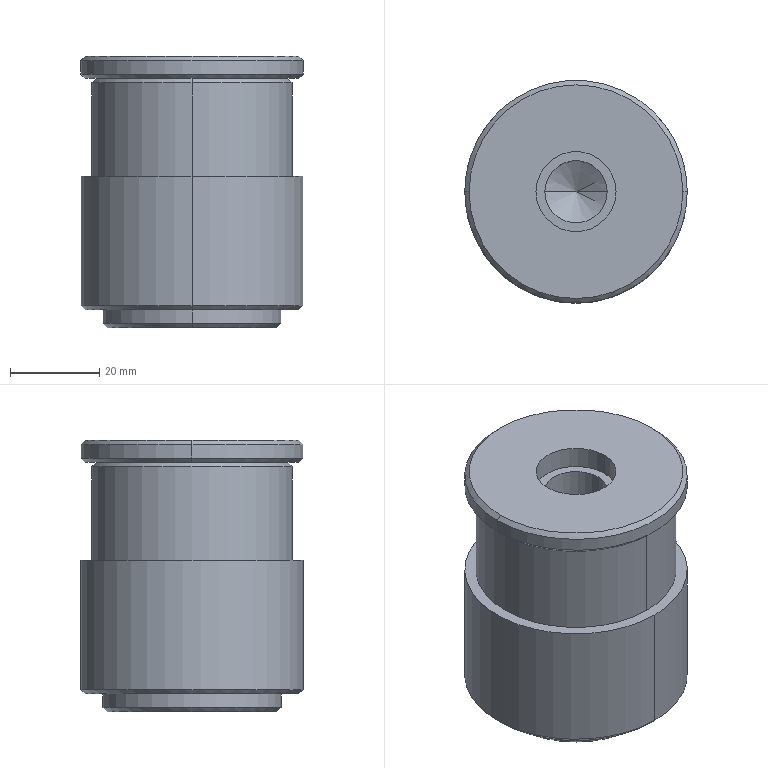Component | SolidWorks | FixedAxis1-1 | 2 solids | 30 faces | box 50 x 50 x 61 mm | volume 102576 mm3 | cone 12 | cylinder 12 | plane 6 | commonest cylinder face diameters 50 x4 14 x2 45 x2 40 x2 18 x2
build123d program:
from build123d import *

# Parameters (mm, degrees)
M16_TAPPED_HOLE1_D     = 14
M16_TAPPED_HOLE1_DEPTH = 28
M16_TAPPED_HOLE1_TIP   = 4.206
CHAMFER1_SIZE          = 1
SKETCH4_R              = 25
SKETCH4_R_2            = 9
BOSS_EXTRUDE1_DEPTH    = 5
CHAMFER2_SIZE          = 1


with BuildPart() as part:
    # Sketch1 → Revolve1 (revolve)
    with BuildSketch(Plane(origin=(0, 0, 0), x_dir=(0, 0, -1), z_dir=(1, 0, 0)), mode=Mode.PRIVATE) as revolve1_sk:
        Polygon((-28, 0), (28, 0), (28, 20), (24, 20), (24, 25), (-6, 25), (-6, 22.5), (-28, 22.5), align=None)
    revolve(revolve1_sk.sketch.rotate(Axis((0, 0, 28), (0, 0, -1)), 180), axis=Axis((0, 0, 28), (0, 0, -1)))

    # M16 Tapped Hole1
    with Locations(Plane.XY.offset(28)):
        with Locations((0, 0)):
            Hole(M16_TAPPED_HOLE1_D / 2, depth=M16_TAPPED_HOLE1_DEPTH)
            with Locations((0, 0, -(M16_TAPPED_HOLE1_DEPTH + M16_TAPPED_HOLE1_TIP / 2))):  # 118° drill point
                Cone(0, M16_TAPPED_HOLE1_D / 2, M16_TAPPED_HOLE1_TIP, mode=Mode.SUBTRACT)

    # Chamfer1
    chamfer1_edges = [part.edges().sort_by_distance(p)[0] for p in [
        (0, 22.5, 28),
        (0, 25, -24),
        (0, 20, -28),
    ]]
    chamfer(chamfer1_edges, length=CHAMFER1_SIZE)


with BuildPart() as body_2:
    # Sketch4 → Boss-Extrude1 (new body)
    with BuildSketch(Plane.XY.offset(28)):
        Circle(SKETCH4_R)
        Circle(SKETCH4_R_2, mode=Mode.SUBTRACT)
    extrude(amount=BOSS_EXTRUDE1_DEPTH)

    # Chamfer2
    chamfer2_edges = [body_2.edges().sort_by_distance(p)[0] for p in [
        (-25, 0, 28),
        (-25, 0, 33),
    ]]
    chamfer(chamfer2_edges, length=CHAMFER2_SIZE)


solid = Compound([part.part, body_2.part])
STEP:
#1=COLOUR_RGB('',0.7922,0.8196,0.9333);
#2=FILL_AREA_STYLE_COLOUR('',#1);
#3=FILL_AREA_STYLE('',(#2));
#4=SURFACE_STYLE_FILL_AREA(#3);
#5=SURFACE_SIDE_STYLE('',(#4));
#6=SURFACE_STYLE_USAGE(.BOTH.,#5);
#7=PRESENTATION_STYLE_ASSIGNMENT((#6));
#8=CARTESIAN_POINT('',(0.,-0.8465,1.102));
#9=VERTEX_POINT('',#8);
#10=CARTESIAN_POINT('',(0.,0.8465,1.102));
#11=VERTEX_POINT('',#10);
#12=CARTESIAN_POINT('',(0.,-0.,1.102));
#13=DIRECTION('',(0.,-0.,1.));
#14=DIRECTION('',(0.,1.,0.));
#15=AXIS2_PLACEMENT_3D('',#12,#13,#14);
#16=CIRCLE('',#15,0.8465);
#17=EDGE_CURVE('',#9,#11,#16,.T.);
#18=ORIENTED_EDGE('',*,*,#17,.F.);
#19=CARTESIAN_POINT('',(0.,-0.8858,1.063));
#20=VERTEX_POINT('',#19);
#21=CARTESIAN_POINT('',(0.,-0.8465,1.102));
#22=DIRECTION('',(0.,-0.7071,-0.7071));
#23=VECTOR('',#22,39.37);
#24=LINE('',#21,#23);
#25=EDGE_CURVE('',#9,#20,#24,.T.);
#26=ORIENTED_EDGE('',*,*,#25,.T.);
#27=CARTESIAN_POINT('',(0.,0.8858,1.063));
#28=VERTEX_POINT('',#27);
#29=CARTESIAN_POINT('',(0.,-0.,1.063));
#30=DIRECTION('',(0.,0.,-1.));
#31=DIRECTION('',(0.,1.,0.));
#32=AXIS2_PLACEMENT_3D('',#29,#30,#31);
#33=CIRCLE('',#32,0.8858);
#34=EDGE_CURVE('',#28,#20,#33,.T.);
#35=ORIENTED_EDGE('',*,*,#34,.F.);
#36=CARTESIAN_POINT('',(0.,0.8465,1.102));
#37=DIRECTION('',(0.,0.7071,-0.7071));
#38=VECTOR('',#37,39.37);
#39=LINE('',#36,#38);
#40=EDGE_CURVE('',#11,#28,#39,.T.);
#41=ORIENTED_EDGE('',*,*,#40,.F.);
#42=EDGE_LOOP('',(#18,#26,#35,#41));
#43=FACE_OUTER_BOUND('',#42,.T.);
#44=CARTESIAN_POINT('',(0.,-0.,1.102));
#45=DIRECTION('',(0.,0.,-1.));
#46=DIRECTION('',(0.,1.,0.));
#47=AXIS2_PLACEMENT_3D('',#44,#45,#46);
#48=CONICAL_SURFACE('',#47,0.8465,0.7854);
#49=ADVANCED_FACE('',(#43),#48,.T.);
#50=CARTESIAN_POINT('',(0.,0.748,-1.102));
#51=VERTEX_POINT('',#50);
#52=CARTESIAN_POINT('',(0.,-0.748,-1.102));
#53=VERTEX_POINT('',#52);
#54=CARTESIAN_POINT('',(0.,-0.,-1.102));
#55=DIRECTION('',(0.,0.,-1.));
#56=DIRECTION('',(0.,-1.,-0.));
#57=AXIS2_PLACEMENT_3D('',#54,#55,#56);
#58=CIRCLE('',#57,0.748);
#59=EDGE_CURVE('',#51,#53,#58,.T.);
#60=ORIENTED_EDGE('',*,*,#59,.F.);
#61=CARTESIAN_POINT('',(0.,0.7874,-1.063));
#62=VERTEX_POINT('',#61);
#63=CARTESIAN_POINT('',(0.,0.7874,-1.063));
#64=DIRECTION('',(0.,0.7071,0.7071));
#65=VECTOR('',#64,39.37);
#66=LINE('',#63,#65);
#67=EDGE_CURVE('',#51,#62,#66,.T.);
#68=ORIENTED_EDGE('',*,*,#67,.T.);
#69=CARTESIAN_POINT('',(0.,-0.7874,-1.063));
#70=VERTEX_POINT('',#69);
#71=CARTESIAN_POINT('',(0.,-0.,-1.063));
#72=DIRECTION('',(0.,-0.,1.));
#73=DIRECTION('',(0.,-1.,-0.));
#74=AXIS2_PLACEMENT_3D('',#71,#72,#73);
#75=CIRCLE('',#74,0.7874);
#76=EDGE_CURVE('',#70,#62,#75,.T.);
#77=ORIENTED_EDGE('',*,*,#76,.F.);
#78=CARTESIAN_POINT('',(0.,-0.7874,-1.063));
#79=DIRECTION('',(0.,-0.7071,0.7071));
#80=VECTOR('',#79,39.37);
#81=LINE('',#78,#80);
#82=EDGE_CURVE('',#53,#70,#81,.T.);
#83=ORIENTED_EDGE('',*,*,#82,.F.);
#84=EDGE_LOOP('',(#60,#68,#77,#83));
#85=FACE_OUTER_BOUND('',#84,.T.);
#86=CARTESIAN_POINT('',(0.,-0.,-1.063));
#87=DIRECTION('',(0.,-0.,1.));
#88=DIRECTION('',(0.,-1.,-0.));
#89=AXIS2_PLACEMENT_3D('',#86,#87,#88);
#90=CONICAL_SURFACE('',#89,0.7874,0.7854);
#91=ADVANCED_FACE('',(#85),#90,.T.);
#92=CARTESIAN_POINT('',(0.,0.9449,-0.9449));
#93=VERTEX_POINT('',#92);
#94=CARTESIAN_POINT('',(0.,-0.9449,-0.9449));
#95=VERTEX_POINT('',#94);
#96=CARTESIAN_POINT('',(0.,-0.,-0.9449));
#97=DIRECTION('',(0.,0.,-1.));
#98=DIRECTION('',(0.,-1.,-0.));
#99=AXIS2_PLACEMENT_3D('',#96,#97,#98);
#100=CIRCLE('',#99,0.9449);
#101=EDGE_CURVE('',#93,#95,#100,.T.);
#102=ORIENTED_EDGE('',*,*,#101,.F.);
#103=CARTESIAN_POINT('',(0.,0.9843,-0.9055));
#104=VERTEX_POINT('',#103);
#105=CARTESIAN_POINT('',(0.,0.9843,-0.9055));
#106=DIRECTION('',(0.,0.7071,0.7071));
#107=VECTOR('',#106,39.37);
#108=LINE('',#105,#107);
#109=EDGE_CURVE('',#93,#104,#108,.T.);
#110=ORIENTED_EDGE('',*,*,#109,.T.);
#111=CARTESIAN_POINT('',(0.,-0.9843,-0.9055));
#112=VERTEX_POINT('',#111);
#113=CARTESIAN_POINT('',(0.,-0.,-0.9055));
#114=DIRECTION('',(0.,-0.,1.));
#115=DIRECTION('',(0.,-1.,-0.));
#116=AXIS2_PLACEMENT_3D('',#113,#114,#115);
#117=CIRCLE('',#116,0.9843);
#118=EDGE_CURVE('',#112,#104,#117,.T.);
#119=ORIENTED_EDGE('',*,*,#118,.F.);
#120=CARTESIAN_POINT('',(0.,-0.9843,-0.9055));
#121=DIRECTION('',(0.,-0.7071,0.7071));
#122=VECTOR('',#121,39.37);
#123=LINE('',#120,#122);
#124=EDGE_CURVE('',#95,#112,#123,.T.);
#125=ORIENTED_EDGE('',*,*,#124,.F.);
#126=EDGE_LOOP('',(#102,#110,#119,#125));
#127=FACE_OUTER_BOUND('',#126,.T.);
#128=CARTESIAN_POINT('',(0.,-0.,-0.9055));
#129=DIRECTION('',(0.,-0.,1.));
#130=DIRECTION('',(0.,-1.,-0.));
#131=AXIS2_PLACEMENT_3D('',#128,#129,#130);
#132=CONICAL_SURFACE('',#131,0.9843,0.7854);
#133=ADVANCED_FACE('',(#127),#132,.T.);
#134=CARTESIAN_POINT('',(-0.2756,0.,-0.));
#135=VERTEX_POINT('',#134);
#136=CARTESIAN_POINT('',(0.2756,0.,-0.));
#137=VERTEX_POINT('',#136);
#138=CARTESIAN_POINT('',(0.,0.,-0.));
#139=DIRECTION('',(0.,0.,1.));
#140=DIRECTION('',(1.,0.,0.));
#141=AXIS2_PLACEMENT_3D('',#138,#139,#140);
#142=CIRCLE('',#141,0.2756);
#143=EDGE_CURVE('',#135,#137,#142,.T.);
#144=ORIENTED_EDGE('',*,*,#143,.F.);
#145=CARTESIAN_POINT('',(-0.2756,0.,1.102));
#146=VERTEX_POINT('',#145);
#147=CARTESIAN_POINT('',(-0.2756,0.,1.102));
#148=DIRECTION('',(0.,0.,1.));
#149=VECTOR('',#148,39.37);
#150=LINE('',#147,#149);
#151=EDGE_CURVE('',#135,#146,#150,.T.);
#152=ORIENTED_EDGE('',*,*,#151,.T.);
#153=CARTESIAN_POINT('',(0.2756,0.,1.102));
#154=VERTEX_POINT('',#153);
#155=CARTESIAN_POINT('',(0.,0.,1.102));
#156=DIRECTION('',(0.,0.,1.));
#157=DIRECTION('',(1.,0.,0.));
#158=AXIS2_PLACEMENT_3D('',#155,#156,#157);
#159=CIRCLE('',#158,0.2756);
#160=EDGE_CURVE('',#146,#154,#159,.T.);
#161=ORIENTED_EDGE('',*,*,#160,.T.);
#162=CARTESIAN_POINT('',(0.2756,0.,1.102));
#163=DIRECTION('',(0.,0.,1.));
#164=VECTOR('',#163,39.37);
#165=LINE('',#162,#164);
#166=EDGE_CURVE('',#137,#154,#165,.T.);
#167=ORIENTED_EDGE('',*,*,#166,.F.);
#168=EDGE_LOOP('',(#144,#152,#161,#167));
#169=FACE_OUTER_BOUND('',#168,.T.);
#170=CARTESIAN_POINT('',(0.,0.,1.102));
#171=DIRECTION('',(0.,0.,1.));
#172=DIRECTION('',(1.,0.,0.));
#173=AXIS2_PLACEMENT_3D('',#170,#171,#172);
#174=CYLINDRICAL_SURFACE('',#173,0.2756);
#175=ADVANCED_FACE('',(#169),#174,.F.);
#176=CARTESIAN_POINT('',(-0.,0.,-0.1656));
#177=VERTEX_POINT('',#176);
#178=CARTESIAN_POINT('',(0.2756,0.,-0.));
#179=DIRECTION('',(0.8572,0.,0.515));
#180=VECTOR('',#179,39.37);
#181=LINE('',#178,#180);
#182=EDGE_CURVE('',#177,#137,#181,.T.);
#183=ORIENTED_EDGE('',*,*,#182,.F.);
#184=CARTESIAN_POINT('',(-0.2756,0.,-0.));
#185=DIRECTION('',(-0.8572,0.,0.515));
#186=VECTOR('',#185,39.37);
#187=LINE('',#184,#186);
#188=EDGE_CURVE('',#177,#135,#187,.T.);
#189=ORIENTED_EDGE('',*,*,#188,.T.);
#190=ORIENTED_EDGE('',*,*,#143,.T.);
#191=EDGE_LOOP('',(#183,#189,#190));
#192=FACE_OUTER_BOUND('',#191,.T.);
#193=CARTESIAN_POINT('',(0.,0.,-0.));
#194=DIRECTION('',(0.,0.,1.));
#195=DIRECTION('',(1.,0.,0.));
#196=AXIS2_PLACEMENT_3D('',#193,#194,#195);
#197=CONICAL_SURFACE('',#196,0.2756,1.03);
#198=ADVANCED_FACE('',(#192),#197,.F.);
#199=CARTESIAN_POINT('',(0.,-0.8858,0.2362));
#200=VERTEX_POINT('',#199);
#201=CARTESIAN_POINT('',(0.,0.8858,0.2362));
#202=VERTEX_POINT('',#201);
#203=CARTESIAN_POINT('',(0.,-0.,0.2362));
#204=DIRECTION('',(0.,-0.,1.));
#205=DIRECTION('',(0.,-1.,-0.));
#206=AXIS2_PLACEMENT_3D('',#203,#204,#205);
#207=CIRCLE('',#206,0.8858);
#208=EDGE_CURVE('',#200,#202,#207,.T.);
#209=ORIENTED_EDGE('',*,*,#208,.T.);
#210=CARTESIAN_POINT('',(0.,0.8858,1.102));
#211=DIRECTION('',(0.,-0.,1.));
#212=VECTOR('',#211,39.37);
#213=LINE('',#210,#212);
#214=EDGE_CURVE('',#202,#28,#213,.T.);
#215=ORIENTED_EDGE('',*,*,#214,.T.);
#216=ORIENTED_EDGE('',*,*,#34,.T.);
#217=CARTESIAN_POINT('',(0.,-0.8858,1.102));
#218=DIRECTION('',(0.,-0.,1.));
#219=VECTOR('',#218,39.37);
#220=LINE('',#217,#219);
#221=EDGE_CURVE('',#200,#20,#220,.T.);
#222=ORIENTED_EDGE('',*,*,#221,.F.);
#223=EDGE_LOOP('',(#209,#215,#216,#222));
#224=FACE_OUTER_BOUND('',#223,.T.);
#225=CARTESIAN_POINT('',(0.,-0.,1.102));
#226=DIRECTION('',(0.,-0.,1.));
#227=DIRECTION('',(0.,-1.,-0.));
#228=AXIS2_PLACEMENT_3D('',#225,#226,#227);
#229=CYLINDRICAL_SURFACE('',#228,0.8858);
#230=ADVANCED_FACE('',(#224),#229,.T.);
#231=ORIENTED_EDGE('',*,*,#118,.T.);
#232=CARTESIAN_POINT('',(0.,0.9843,0.2362));
#233=VERTEX_POINT('',#232);
#234=CARTESIAN_POINT('',(0.,0.9843,1.102));
#235=DIRECTION('',(0.,-0.,1.));
#236=VECTOR('',#235,39.37);
#237=LINE('',#234,#236);
#238=EDGE_CURVE('',#104,#233,#237,.T.);
#239=ORIENTED_EDGE('',*,*,#238,.T.);
#240=CARTESIAN_POINT('',(0.,-0.9843,0.2362));
#241=VERTEX_POINT('',#240);
#242=CARTESIAN_POINT('',(0.,-0.,0.2362));
#243=DIRECTION('',(0.,-0.,1.));
#244=DIRECTION('',(0.,-1.,-0.));
#245=AXIS2_PLACEMENT_3D('',#242,#243,#244);
#246=CIRCLE('',#245,0.9843);
#247=EDGE_CURVE('',#241,#233,#246,.T.);
#248=ORIENTED_EDGE('',*,*,#247,.F.);
#249=CARTESIAN_POINT('',(0.,-0.9843,1.102));
#250=DIRECTION('',(0.,-0.,1.));
#251=VECTOR('',#250,39.37);
#252=LINE('',#249,#251);
#253=EDGE_CURVE('',#112,#241,#252,.T.);
#254=ORIENTED_EDGE('',*,*,#253,.F.);
#255=EDGE_LOOP('',(#231,#239,#248,#254));
#256=FACE_OUTER_BOUND('',#255,.T.);
#257=CARTESIAN_POINT('',(0.,-0.,1.102));
#258=DIRECTION('',(0.,-0.,1.));
#259=DIRECTION('',(0.,-1.,-0.));
#260=AXIS2_PLACEMENT_3D('',#257,#258,#259);
#261=CYLINDRICAL_SURFACE('',#260,0.9843);
#262=ADVANCED_FACE('',(#256),#261,.T.);
#263=ORIENTED_EDGE('',*,*,#76,.T.);
#264=CARTESIAN_POINT('',(0.,0.7874,-0.9449));
#265=VERTEX_POINT('',#264);
#266=CARTESIAN_POINT('',(0.,0.7874,1.102));
#267=DIRECTION('',(0.,-0.,1.));
#268=VECTOR('',#267,39.37);
#269=LINE('',#266,#268);
#270=EDGE_CURVE('',#62,#265,#269,.T.);
#271=ORIENTED_EDGE('',*,*,#270,.T.);
#272=CARTESIAN_POINT('',(0.,-0.7874,-0.9449));
#273=VERTEX_POINT('',#272);
#274=CARTESIAN_POINT('',(0.,-0.,-0.9449));
#275=DIRECTION('',(0.,-0.,1.));
#276=DIRECTION('',(0.,-1.,-0.));
#277=AXIS2_PLACEMENT_3D('',#274,#275,#276);
#278=CIRCLE('',#277,0.7874);
#279=EDGE_CURVE('',#273,#265,#278,.T.);
#280=ORIENTED_EDGE('',*,*,#279,.F.);
#281=CARTESIAN_POINT('',(0.,-0.7874,1.102));
#282=DIRECTION('',(0.,-0.,1.));
#283=VECTOR('',#282,39.37);
#284=LINE('',#281,#283);
#285=EDGE_CURVE('',#70,#273,#284,.T.);
#286=ORIENTED_EDGE('',*,*,#285,.F.);
#287=EDGE_LOOP('',(#263,#271,#280,#286));
#288=FACE_OUTER_BOUND('',#287,.T.);
#289=CARTESIAN_POINT('',(0.,-0.,1.102));
#290=DIRECTION('',(0.,-0.,1.));
#291=DIRECTION('',(0.,-1.,-0.));
#292=AXIS2_PLACEMENT_3D('',#289,#290,#291);
#293=CYLINDRICAL_SURFACE('',#292,0.7874);
#294=ADVANCED_FACE('',(#288),#293,.T.);
#295=CARTESIAN_POINT('',(0.,-0.,1.102));
#296=DIRECTION('',(0.,-0.,1.));
#297=DIRECTION('',(0.,1.,0.));
#298=AXIS2_PLACEMENT_3D('',#295,#296,#297);
#299=CIRCLE('',#298,0.8465);
#300=EDGE_CURVE('',#11,#9,#299,.T.);
#301=ORIENTED_EDGE('',*,*,#300,.T.);
#302=ORIENTED_EDGE('',*,*,#17,.T.);
#303=EDGE_LOOP('',(#301,#302));
#304=FACE_OUTER_BOUND('',#303,.T.);
#305=CARTESIAN_POINT('',(0.,0.,1.102));
#306=DIRECTION('',(0.,0.,1.));
#307=DIRECTION('',(1.,0.,0.));
#308=AXIS2_PLACEMENT_3D('',#305,#306,#307);
#309=CIRCLE('',#308,0.2756);
#310=EDGE_CURVE('',#154,#146,#309,.T.);
#311=ORIENTED_EDGE('',*,*,#310,.F.);
#312=ORIENTED_EDGE('',*,*,#160,.F.);
#313=EDGE_LOOP('',(#311,#312));
#314=FACE_BOUND('',#313,.T.);
#315=CARTESIAN_POINT('',(0.,0.8858,1.102));
#316=DIRECTION('',(0.,0.,-1.));
#317=DIRECTION('',(0.,1.,0.));
#318=AXIS2_PLACEMENT_3D('',#315,#316,#317);
#319=PLANE('',#318);
#320=ADVANCED_FACE('',(#304,#314),#319,.F.);
#321=CARTESIAN_POINT('',(0.,-0.,-1.102));
#322=DIRECTION('',(0.,0.,-1.));
#323=DIRECTION('',(0.,-1.,-0.));
#324=AXIS2_PLACEMENT_3D('',#321,#322,#323);
#325=CIRCLE('',#324,0.748);
#326=EDGE_CURVE('',#53,#51,#325,.T.);
#327=ORIENTED_EDGE('',*,*,#326,.T.);
#328=ORIENTED_EDGE('',*,*,#59,.T.);
#329=EDGE_LOOP('',(#327,#328));
#330=FACE_OUTER_BOUND('',#329,.T.);
#331=CARTESIAN_POINT('',(0.,-0.,-1.102));
#332=DIRECTION('',(0.,-0.,1.));
#333=DIRECTION('',(0.,-1.,-0.));
#334=AXIS2_PLACEMENT_3D('',#331,#332,#333);
#335=PLANE('',#334);
#336=ADVANCED_FACE('',(#330),#335,.F.);
#337=ORIENTED_EDGE('',*,*,#270,.F.);
#338=CARTESIAN_POINT('',(0.,-0.,-1.063));
#339=DIRECTION('',(0.,-0.,1.));
#340=DIRECTION('',(0.,-1.,-0.));
#341=AXIS2_PLACEMENT_3D('',#338,#339,#340);
#342=CIRCLE('',#341,0.7874);
#343=EDGE_CURVE('',#62,#70,#342,.T.);
#344=ORIENTED_EDGE('',*,*,#343,.T.);
#345=ORIENTED_EDGE('',*,*,#285,.T.);
#346=CARTESIAN_POINT('',(0.,-0.,-0.9449));
#347=DIRECTION('',(0.,-0.,1.));
#348=DIRECTION('',(0.,-1.,-0.));
#349=AXIS2_PLACEMENT_3D('',#346,#347,#348);
#350=CIRCLE('',#349,0.7874);
#351=EDGE_CURVE('',#265,#273,#350,.T.);
#352=ORIENTED_EDGE('',*,*,#351,.F.);
#353=EDGE_LOOP('',(#337,#344,#345,#352));
#354=FACE_OUTER_BOUND('',#353,.T.);
#355=CARTESIAN_POINT('',(0.,-0.,1.102));
#356=DIRECTION('',(0.,-0.,1.));
#357=DIRECTION('',(0.,-1.,-0.));
#358=AXIS2_PLACEMENT_3D('',#355,#356,#357);
#359=CYLINDRICAL_SURFACE('',#358,0.7874);
#360=ADVANCED_FACE('',(#354),#359,.T.);
#361=CARTESIAN_POINT('',(0.,-0.,-0.9449));
#362=DIRECTION('',(0.,0.,-1.));
#363=DIRECTION('',(0.,-1.,-0.));
#364=AXIS2_PLACEMENT_3D('',#361,#362,#363);
#365=CIRCLE('',#364,0.9449);
#366=EDGE_CURVE('',#95,#93,#365,.T.);
#367=ORIENTED_EDGE('',*,*,#366,.T.);
#368=ORIENTED_EDGE('',*,*,#101,.T.);
#369=EDGE_LOOP('',(#367,#368));
#370=FACE_OUTER_BOUND('',#369,.T.);
#371=ORIENTED_EDGE('',*,*,#279,.T.);
#372=ORIENTED_EDGE('',*,*,#351,.T.);
#373=EDGE_LOOP('',(#371,#372));
#374=FACE_BOUND('',#373,.T.);
#375=CARTESIAN_POINT('',(0.,0.7874,-0.9449));
#376=DIRECTION('',(0.,-0.,1.));
#377=DIRECTION('',(0.,-1.,-0.));
#378=AXIS2_PLACEMENT_3D('',#375,#376,#377);
#379=PLANE('',#378);
#380=ADVANCED_FACE('',(#370,#374),#379,.F.);
#381=ORIENTED_EDGE('',*,*,#238,.F.);
#382=CARTESIAN_POINT('',(0.,-0.,-0.9055));
#383=DIRECTION('',(0.,-0.,1.));
#384=DIRECTION('',(0.,-1.,-0.));
#385=AXIS2_PLACEMENT_3D('',#382,#383,#384);
#386=CIRCLE('',#385,0.9843);
#387=EDGE_CURVE('',#104,#112,#386,.T.);
#388=ORIENTED_EDGE('',*,*,#387,.T.);
#389=ORIENTED_EDGE('',*,*,#253,.T.);
#390=CARTESIAN_POINT('',(0.,-0.,0.2362));
#391=DIRECTION('',(0.,-0.,1.));
#392=DIRECTION('',(0.,-1.,-0.));
#393=AXIS2_PLACEMENT_3D('',#390,#391,#392);
#394=CIRCLE('',#393,0.9843);
#395=EDGE_CURVE('',#233,#241,#394,.T.);
#396=ORIENTED_EDGE('',*,*,#395,.F.);
#397=EDGE_LOOP('',(#381,#388,#389,#396));
#398=FACE_OUTER_BOUND('',#397,.T.);
#399=CARTESIAN_POINT('',(0.,-0.,1.102));
#400=DIRECTION('',(0.,-0.,1.));
#401=DIRECTION('',(0.,-1.,-0.));
#402=AXIS2_PLACEMENT_3D('',#399,#400,#401);
#403=CYLINDRICAL_SURFACE('',#402,0.9843);
#404=ADVANCED_FACE('',(#398),#403,.T.);
#405=ORIENTED_EDGE('',*,*,#208,.F.);
#406=CARTESIAN_POINT('',(0.,-0.,0.2362));
#407=DIRECTION('',(0.,-0.,1.));
#408=DIRECTION('',(0.,-1.,-0.));
#409=AXIS2_PLACEMENT_3D('',#406,#407,#408);
#410=CIRCLE('',#409,0.8858);
#411=EDGE_CURVE('',#202,#200,#410,.T.);
#412=ORIENTED_EDGE('',*,*,#411,.F.);
#413=EDGE_LOOP('',(#405,#412));
#414=FACE_BOUND('',#413,.T.);
#415=ORIENTED_EDGE('',*,*,#247,.T.);
#416=ORIENTED_EDGE('',*,*,#395,.T.);
#417=EDGE_LOOP('',(#415,#416));
#418=FACE_OUTER_BOUND('',#417,.T.);
#419=CARTESIAN_POINT('',(0.,0.9843,0.2362));
#420=DIRECTION('',(0.,0.,-1.));
#421=DIRECTION('',(0.,1.,0.));
#422=AXIS2_PLACEMENT_3D('',#419,#420,#421);
#423=PLANE('',#422);
#424=ADVANCED_FACE('',(#414,#418),#423,.F.);
#425=ORIENTED_EDGE('',*,*,#214,.F.);
#426=ORIENTED_EDGE('',*,*,#411,.T.);
#427=ORIENTED_EDGE('',*,*,#221,.T.);
#428=CARTESIAN_POINT('',(0.,-0.,1.063));
#429=DIRECTION('',(0.,0.,-1.));
#430=DIRECTION('',(0.,1.,0.));
#431=AXIS2_PLACEMENT_3D('',#428,#429,#430);
#432=CIRCLE('',#431,0.8858);
#433=EDGE_CURVE('',#20,#28,#432,.T.);
#434=ORIENTED_EDGE('',*,*,#433,.T.);
#435=EDGE_LOOP('',(#425,#426,#427,#434));
#436=FACE_OUTER_BOUND('',#435,.T.);
#437=CARTESIAN_POINT('',(0.,-0.,1.102));
#438=DIRECTION('',(0.,-0.,1.));
#439=DIRECTION('',(0.,-1.,-0.));
#440=AXIS2_PLACEMENT_3D('',#437,#438,#439);
#441=CYLINDRICAL_SURFACE('',#440,0.8858);
#442=ADVANCED_FACE('',(#436),#441,.T.);
#443=ORIENTED_EDGE('',*,*,#188,.F.);
#444=ORIENTED_EDGE('',*,*,#182,.T.);
#445=CARTESIAN_POINT('',(0.,0.,-0.));
#446=DIRECTION('',(0.,0.,1.));
#447=DIRECTION('',(1.,0.,0.));
#448=AXIS2_PLACEMENT_3D('',#445,#446,#447);
#449=CIRCLE('',#448,0.2756);
#450=EDGE_CURVE('',#137,#135,#449,.T.);
#451=ORIENTED_EDGE('',*,*,#450,.T.);
#452=EDGE_LOOP('',(#443,#444,#451));
#453=FACE_OUTER_BOUND('',#452,.T.);
#454=CARTESIAN_POINT('',(0.,0.,-0.));
#455=DIRECTION('',(0.,0.,1.));
#456=DIRECTION('',(1.,0.,0.));
#457=AXIS2_PLACEMENT_3D('',#454,#455,#456);
#458=CONICAL_SURFACE('',#457,0.2756,1.03);
#459=ADVANCED_FACE('',(#453),#458,.F.);
#460=ORIENTED_EDGE('',*,*,#151,.F.);
#461=ORIENTED_EDGE('',*,*,#450,.F.);
#462=ORIENTED_EDGE('',*,*,#166,.T.);
#463=ORIENTED_EDGE('',*,*,#310,.T.);
#464=EDGE_LOOP('',(#460,#461,#462,#463));
#465=FACE_OUTER_BOUND('',#464,.T.);
#466=CARTESIAN_POINT('',(0.,0.,1.102));
#467=DIRECTION('',(0.,0.,1.));
#468=DIRECTION('',(1.,0.,0.));
#469=AXIS2_PLACEMENT_3D('',#466,#467,#468);
#470=CYLINDRICAL_SURFACE('',#469,0.2756);
#471=ADVANCED_FACE('',(#465),#470,.F.);
#472=ORIENTED_EDGE('',*,*,#109,.F.);
#473=ORIENTED_EDGE('',*,*,#366,.F.);
#474=ORIENTED_EDGE('',*,*,#124,.T.);
#475=ORIENTED_EDGE('',*,*,#387,.F.);
#476=EDGE_LOOP('',(#472,#473,#474,#475));
#477=FACE_OUTER_BOUND('',#476,.T.);
#478=CARTESIAN_POINT('',(0.,-0.,-0.9055));
#479=DIRECTION('',(0.,-0.,1.));
#480=DIRECTION('',(0.,-1.,-0.));
#481=AXIS2_PLACEMENT_3D('',#478,#479,#480);
#482=CONICAL_SURFACE('',#481,0.9843,0.7854);
#483=ADVANCED_FACE('',(#477),#482,.T.);
#484=ORIENTED_EDGE('',*,*,#67,.F.);
#485=ORIENTED_EDGE('',*,*,#326,.F.);
#486=ORIENTED_EDGE('',*,*,#82,.T.);
#487=ORIENTED_EDGE('',*,*,#343,.F.);
#488=EDGE_LOOP('',(#484,#485,#486,#487));
#489=FACE_OUTER_BOUND('',#488,.T.);
#490=CARTESIAN_POINT('',(0.,-0.,-1.063));
#491=DIRECTION('',(0.,-0.,1.));
#492=DIRECTION('',(0.,-1.,-0.));
#493=AXIS2_PLACEMENT_3D('',#490,#491,#492);
#494=CONICAL_SURFACE('',#493,0.7874,0.7854);
#495=ADVANCED_FACE('',(#489),#494,.T.);
#496=ORIENTED_EDGE('',*,*,#25,.F.);
#497=ORIENTED_EDGE('',*,*,#300,.F.);
#498=ORIENTED_EDGE('',*,*,#40,.T.);
#499=ORIENTED_EDGE('',*,*,#433,.F.);
#500=EDGE_LOOP('',(#496,#497,#498,#499));
#501=FACE_OUTER_BOUND('',#500,.T.);
#502=CARTESIAN_POINT('',(0.,-0.,1.102));
#503=DIRECTION('',(0.,0.,-1.));
#504=DIRECTION('',(0.,1.,0.));
#505=AXIS2_PLACEMENT_3D('',#502,#503,#504);
#506=CONICAL_SURFACE('',#505,0.8465,0.7854);
#507=ADVANCED_FACE('',(#501),#506,.T.);
#508=CLOSED_SHELL('',(#49,#91,#133,#175,#198,#230,#262,#294,#320,#336,#360,#380,#404,#424,#442,#459,#471,#483,#495,#507));
#509=MANIFOLD_SOLID_BREP('',#508);
#510=STYLED_ITEM('',(#7),#509);
#511=PRESENTATION_LAYER_ASSIGNMENT('','',(#510));
#512=(LENGTH_UNIT()NAMED_UNIT(*)SI_UNIT($,.METRE.));
#513=LENGTH_MEASURE_WITH_UNIT(LENGTH_MEASURE(0.0254),#512);
#514=DIMENSIONAL_EXPONENTS(1.,0.,0.,0.,0.,0.,0.);
#515=(CONVERSION_BASED_UNIT('',#513)LENGTH_UNIT()NAMED_UNIT(#514));
#516=UNCERTAINTY_MEASURE_WITH_UNIT(LENGTH_MEASURE(0.00001),#515,'','');
#517=(NAMED_UNIT(*)PLANE_ANGLE_UNIT()SI_UNIT($,.RADIAN.));
#518=(NAMED_UNIT(*)SI_UNIT($,.STERADIAN.)SOLID_ANGLE_UNIT());
#519=(GEOMETRIC_REPRESENTATION_CONTEXT(3)GLOBAL_UNCERTAINTY_ASSIGNED_CONTEXT((#516))GLOBAL_UNIT_ASSIGNED_CONTEXT((#515,#517,#518))REPRESENTATION_CONTEXT('',''));
#520=MECHANICAL_DESIGN_GEOMETRIC_PRESENTATION_REPRESENTATION('',(#510),#519);
#521=COLOUR_RGB('',0.7922,0.8196,0.9333);
#522=FILL_AREA_STYLE_COLOUR('',#521);
#523=FILL_AREA_STYLE('',(#522));
#524=SURFACE_STYLE_FILL_AREA(#523);
#525=SURFACE_SIDE_STYLE('',(#524));
#526=SURFACE_STYLE_USAGE(.BOTH.,#525);
#527=PRESENTATION_STYLE_ASSIGNMENT((#526));
#528=CARTESIAN_POINT('',(0.9449,0.,1.299));
#529=VERTEX_POINT('',#528);
#530=CARTESIAN_POINT('',(-0.9449,0.,1.299));
#531=VERTEX_POINT('',#530);
#532=CARTESIAN_POINT('',(0.,0.,1.299));
#533=DIRECTION('',(0.,0.,1.));
#534=DIRECTION('',(1.,0.,0.));
#535=AXIS2_PLACEMENT_3D('',#532,#533,#534);
#536=CIRCLE('',#535,0.9449);
#537=EDGE_CURVE('',#529,#531,#536,.T.);
#538=ORIENTED_EDGE('',*,*,#537,.F.);
#539=CARTESIAN_POINT('',(0.9843,0.,1.26));
#540=VERTEX_POINT('',#539);
#541=CARTESIAN_POINT('',(0.9449,0.,1.299));
#542=DIRECTION('',(0.7071,0.,-0.7071));
#543=VECTOR('',#542,39.37);
#544=LINE('',#541,#543);
#545=EDGE_CURVE('',#529,#540,#544,.T.);
#546=ORIENTED_EDGE('',*,*,#545,.T.);
#547=CARTESIAN_POINT('',(-0.9843,0.,1.26));
#548=VERTEX_POINT('',#547);
#549=CARTESIAN_POINT('',(0.,0.,1.26));
#550=DIRECTION('',(0.,0.,-1.));
#551=DIRECTION('',(1.,0.,0.));
#552=AXIS2_PLACEMENT_3D('',#549,#550,#551);
#553=CIRCLE('',#552,0.9843);
#554=EDGE_CURVE('',#548,#540,#553,.T.);
#555=ORIENTED_EDGE('',*,*,#554,.F.);
#556=CARTESIAN_POINT('',(-0.9449,0.,1.299));
#557=DIRECTION('',(-0.7071,0.,-0.7071));
#558=VECTOR('',#557,39.37);
#559=LINE('',#556,#558);
#560=EDGE_CURVE('',#531,#548,#559,.T.);
#561=ORIENTED_EDGE('',*,*,#560,.F.);
#562=EDGE_LOOP('',(#538,#546,#555,#561));
#563=FACE_OUTER_BOUND('',#562,.T.);
#564=CARTESIAN_POINT('',(0.,0.,1.299));
#565=DIRECTION('',(0.,0.,-1.));
#566=DIRECTION('',(-1.,0.,0.));
#567=AXIS2_PLACEMENT_3D('',#564,#565,#566);
#568=CONICAL_SURFACE('',#567,0.9449,0.7854);
#569=ADVANCED_FACE('',(#563),#568,.T.);
#570=CARTESIAN_POINT('',(-0.9449,0.,1.102));
#571=VERTEX_POINT('',#570);
#572=CARTESIAN_POINT('',(0.9449,0.,1.102));
#573=VERTEX_POINT('',#572);
#574=CARTESIAN_POINT('',(0.,0.,1.102));
#575=DIRECTION('',(0.,0.,-1.));
#576=DIRECTION('',(1.,0.,0.));
#577=AXIS2_PLACEMENT_3D('',#574,#575,#576);
#578=CIRCLE('',#577,0.9449);
#579=EDGE_CURVE('',#571,#573,#578,.T.);
#580=ORIENTED_EDGE('',*,*,#579,.F.);
#581=CARTESIAN_POINT('',(-0.9843,0.,1.142));
#582=VERTEX_POINT('',#581);
#583=CARTESIAN_POINT('',(-0.9843,0.,1.142));
#584=DIRECTION('',(-0.7071,0.,0.7071));
#585=VECTOR('',#584,39.37);
#586=LINE('',#583,#585);
#587=EDGE_CURVE('',#571,#582,#586,.T.);
#588=ORIENTED_EDGE('',*,*,#587,.T.);
#589=CARTESIAN_POINT('',(0.9843,0.,1.142));
#590=VERTEX_POINT('',#589);
#591=CARTESIAN_POINT('',(0.,0.,1.142));
#592=DIRECTION('',(0.,0.,1.));
#593=DIRECTION('',(1.,0.,0.));
#594=AXIS2_PLACEMENT_3D('',#591,#592,#593);
#595=CIRCLE('',#594,0.9843);
#596=EDGE_CURVE('',#590,#582,#595,.T.);
#597=ORIENTED_EDGE('',*,*,#596,.F.);
#598=CARTESIAN_POINT('',(0.9843,0.,1.142));
#599=DIRECTION('',(0.7071,0.,0.7071));
#600=VECTOR('',#599,39.37);
#601=LINE('',#598,#600);
#602=EDGE_CURVE('',#573,#590,#601,.T.);
#603=ORIENTED_EDGE('',*,*,#602,.F.);
#604=EDGE_LOOP('',(#580,#588,#597,#603));
#605=FACE_OUTER_BOUND('',#604,.T.);
#606=CARTESIAN_POINT('',(0.,0.,1.142));
#607=DIRECTION('',(0.,0.,1.));
#608=DIRECTION('',(1.,0.,0.));
#609=AXIS2_PLACEMENT_3D('',#606,#607,#608);
#610=CONICAL_SURFACE('',#609,0.9843,0.7854);
#611=ADVANCED_FACE('',(#605),#610,.T.);
#612=CARTESIAN_POINT('',(-0.3543,0.,1.299));
#613=VERTEX_POINT('',#612);
#614=CARTESIAN_POINT('',(0.3543,0.,1.299));
#615=VERTEX_POINT('',#614);
#616=CARTESIAN_POINT('',(0.,0.,1.299));
#617=DIRECTION('',(0.,0.,1.));
#618=DIRECTION('',(1.,0.,0.));
#619=AXIS2_PLACEMENT_3D('',#616,#617,#618);
#620=CIRCLE('',#619,0.3543);
#621=EDGE_CURVE('',#613,#615,#620,.T.);
#622=ORIENTED_EDGE('',*,*,#621,.T.);
#623=CARTESIAN_POINT('',(0.3543,0.,1.102));
#624=VERTEX_POINT('',#623);
#625=CARTESIAN_POINT('',(0.3543,0.,1.299));
#626=DIRECTION('',(0.,0.,-1.));
#627=VECTOR('',#626,39.37);
#628=LINE('',#625,#627);
#629=EDGE_CURVE('',#615,#624,#628,.T.);
#630=ORIENTED_EDGE('',*,*,#629,.T.);
#631=CARTESIAN_POINT('',(-0.3543,0.,1.102));
#632=VERTEX_POINT('',#631);
#633=CARTESIAN_POINT('',(0.,0.,1.102));
#634=DIRECTION('',(0.,0.,1.));
#635=DIRECTION('',(1.,0.,0.));
#636=AXIS2_PLACEMENT_3D('',#633,#634,#635);
#637=CIRCLE('',#636,0.3543);
#638=EDGE_CURVE('',#632,#624,#637,.T.);
#639=ORIENTED_EDGE('',*,*,#638,.F.);
#640=CARTESIAN_POINT('',(-0.3543,0.,1.299));
#641=DIRECTION('',(0.,0.,-1.));
#642=VECTOR('',#641,39.37);
#643=LINE('',#640,#642);
#644=EDGE_CURVE('',#613,#632,#643,.T.);
#645=ORIENTED_EDGE('',*,*,#644,.F.);
#646=EDGE_LOOP('',(#622,#630,#639,#645));
#647=FACE_OUTER_BOUND('',#646,.T.);
#648=CARTESIAN_POINT('',(0.,0.,1.299));
#649=DIRECTION('',(0.,0.,-1.));
#650=DIRECTION('',(-1.,0.,0.));
#651=AXIS2_PLACEMENT_3D('',#648,#649,#650);
#652=CYLINDRICAL_SURFACE('',#651,0.3543);
#653=ADVANCED_FACE('',(#647),#652,.F.);
#654=ORIENTED_EDGE('',*,*,#554,.T.);
#655=CARTESIAN_POINT('',(0.9843,0.,1.299));
#656=DIRECTION('',(0.,0.,-1.));
#657=VECTOR('',#656,39.37);
#658=LINE('',#655,#657);
#659=EDGE_CURVE('',#540,#590,#658,.T.);
#660=ORIENTED_EDGE('',*,*,#659,.T.);
#661=ORIENTED_EDGE('',*,*,#596,.T.);
#662=CARTESIAN_POINT('',(-0.9843,0.,1.299));
#663=DIRECTION('',(0.,0.,-1.));
#664=VECTOR('',#663,39.37);
#665=LINE('',#662,#664);
#666=EDGE_CURVE('',#548,#582,#665,.T.);
#667=ORIENTED_EDGE('',*,*,#666,.F.);
#668=EDGE_LOOP('',(#654,#660,#661,#667));
#669=FACE_OUTER_BOUND('',#668,.T.);
#670=CARTESIAN_POINT('',(0.,0.,1.299));
#671=DIRECTION('',(0.,0.,-1.));
#672=DIRECTION('',(-1.,0.,0.));
#673=AXIS2_PLACEMENT_3D('',#670,#671,#672);
#674=CYLINDRICAL_SURFACE('',#673,0.9843);
#675=ADVANCED_FACE('',(#669),#674,.T.);
#676=CARTESIAN_POINT('',(0.,0.,1.299));
#677=DIRECTION('',(0.,0.,1.));
#678=DIRECTION('',(1.,0.,0.));
#679=AXIS2_PLACEMENT_3D('',#676,#677,#678);
#680=CIRCLE('',#679,0.9449);
#681=EDGE_CURVE('',#531,#529,#680,.T.);
#682=ORIENTED_EDGE('',*,*,#681,.T.);
#683=ORIENTED_EDGE('',*,*,#537,.T.);
#684=EDGE_LOOP('',(#682,#683));
#685=FACE_OUTER_BOUND('',#684,.T.);
#686=ORIENTED_EDGE('',*,*,#621,.F.);
#687=CARTESIAN_POINT('',(0.,0.,1.299));
#688=DIRECTION('',(0.,0.,1.));
#689=DIRECTION('',(1.,0.,0.));
#690=AXIS2_PLACEMENT_3D('',#687,#688,#689);
#691=CIRCLE('',#690,0.3543);
#692=EDGE_CURVE('',#615,#613,#691,.T.);
#693=ORIENTED_EDGE('',*,*,#692,.F.);
#694=EDGE_LOOP('',(#686,#693));
#695=FACE_BOUND('',#694,.T.);
#696=CARTESIAN_POINT('',(0.,0.,1.299));
#697=DIRECTION('',(0.,0.,1.));
#698=DIRECTION('',(1.,0.,0.));
#699=AXIS2_PLACEMENT_3D('',#696,#697,#698);
#700=PLANE('',#699);
#701=ADVANCED_FACE('',(#685,#695),#700,.T.);
#702=CARTESIAN_POINT('',(0.,0.,1.102));
#703=DIRECTION('',(0.,0.,-1.));
#704=DIRECTION('',(1.,0.,0.));
#705=AXIS2_PLACEMENT_3D('',#702,#703,#704);
#706=CIRCLE('',#705,0.9449);
#707=EDGE_CURVE('',#573,#571,#706,.T.);
#708=ORIENTED_EDGE('',*,*,#707,.T.);
#709=ORIENTED_EDGE('',*,*,#579,.T.);
#710=EDGE_LOOP('',(#708,#709));
#711=FACE_OUTER_BOUND('',#710,.T.);
#712=ORIENTED_EDGE('',*,*,#638,.T.);
#713=CARTESIAN_POINT('',(0.,0.,1.102));
#714=DIRECTION('',(0.,0.,1.));
#715=DIRECTION('',(1.,0.,0.));
#716=AXIS2_PLACEMENT_3D('',#713,#714,#715);
#717=CIRCLE('',#716,0.3543);
#718=EDGE_CURVE('',#624,#632,#717,.T.);
#719=ORIENTED_EDGE('',*,*,#718,.T.);
#720=EDGE_LOOP('',(#712,#719));
#721=FACE_BOUND('',#720,.T.);
#722=CARTESIAN_POINT('',(0.,0.,1.102));
#723=DIRECTION('',(0.,0.,1.));
#724=DIRECTION('',(1.,0.,0.));
#725=AXIS2_PLACEMENT_3D('',#722,#723,#724);
#726=PLANE('',#725);
#727=ADVANCED_FACE('',(#711,#721),#726,.F.);
#728=ORIENTED_EDGE('',*,*,#659,.F.);
#729=CARTESIAN_POINT('',(0.,0.,1.26));
#730=DIRECTION('',(0.,0.,-1.));
#731=DIRECTION('',(1.,0.,0.));
#732=AXIS2_PLACEMENT_3D('',#729,#730,#731);
#733=CIRCLE('',#732,0.9843);
#734=EDGE_CURVE('',#540,#548,#733,.T.);
#735=ORIENTED_EDGE('',*,*,#734,.T.);
#736=ORIENTED_EDGE('',*,*,#666,.T.);
#737=CARTESIAN_POINT('',(0.,0.,1.142));
#738=DIRECTION('',(0.,0.,1.));
#739=DIRECTION('',(1.,0.,0.));
#740=AXIS2_PLACEMENT_3D('',#737,#738,#739);
#741=CIRCLE('',#740,0.9843);
#742=EDGE_CURVE('',#582,#590,#741,.T.);
#743=ORIENTED_EDGE('',*,*,#742,.T.);
#744=EDGE_LOOP('',(#728,#735,#736,#743));
#745=FACE_OUTER_BOUND('',#744,.T.);
#746=CARTESIAN_POINT('',(0.,0.,1.299));
#747=DIRECTION('',(0.,0.,-1.));
#748=DIRECTION('',(-1.,0.,0.));
#749=AXIS2_PLACEMENT_3D('',#746,#747,#748);
#750=CYLINDRICAL_SURFACE('',#749,0.9843);
#751=ADVANCED_FACE('',(#745),#750,.T.);
#752=ORIENTED_EDGE('',*,*,#629,.F.);
#753=ORIENTED_EDGE('',*,*,#692,.T.);
#754=ORIENTED_EDGE('',*,*,#644,.T.);
#755=ORIENTED_EDGE('',*,*,#718,.F.);
#756=EDGE_LOOP('',(#752,#753,#754,#755));
#757=FACE_OUTER_BOUND('',#756,.T.);
#758=CARTESIAN_POINT('',(0.,0.,1.299));
#759=DIRECTION('',(0.,0.,-1.));
#760=DIRECTION('',(-1.,0.,0.));
#761=AXIS2_PLACEMENT_3D('',#758,#759,#760);
#762=CYLINDRICAL_SURFACE('',#761,0.3543);
#763=ADVANCED_FACE('',(#757),#762,.F.);
#764=ORIENTED_EDGE('',*,*,#587,.F.);
#765=ORIENTED_EDGE('',*,*,#707,.F.);
#766=ORIENTED_EDGE('',*,*,#602,.T.);
#767=ORIENTED_EDGE('',*,*,#742,.F.);
#768=EDGE_LOOP('',(#764,#765,#766,#767));
#769=FACE_OUTER_BOUND('',#768,.T.);
#770=CARTESIAN_POINT('',(0.,0.,1.142));
#771=DIRECTION('',(0.,0.,1.));
#772=DIRECTION('',(1.,0.,0.));
#773=AXIS2_PLACEMENT_3D('',#770,#771,#772);
#774=CONICAL_SURFACE('',#773,0.9843,0.7854);
#775=ADVANCED_FACE('',(#769),#774,.T.);
#776=ORIENTED_EDGE('',*,*,#545,.F.);
#777=ORIENTED_EDGE('',*,*,#681,.F.);
#778=ORIENTED_EDGE('',*,*,#560,.T.);
#779=ORIENTED_EDGE('',*,*,#734,.F.);
#780=EDGE_LOOP('',(#776,#777,#778,#779));
#781=FACE_OUTER_BOUND('',#780,.T.);
#782=CARTESIAN_POINT('',(0.,0.,1.299));
#783=DIRECTION('',(0.,0.,-1.));
#784=DIRECTION('',(-1.,0.,0.));
#785=AXIS2_PLACEMENT_3D('',#782,#783,#784);
#786=CONICAL_SURFACE('',#785,0.9449,0.7854);
#787=ADVANCED_FACE('',(#781),#786,.T.);
#788=CLOSED_SHELL('',(#569,#611,#653,#675,#701,#727,#751,#763,#775,#787));
#789=MANIFOLD_SOLID_BREP('',#788);
#790=STYLED_ITEM('',(#527),#789);
#791=(LENGTH_UNIT()NAMED_UNIT(*)SI_UNIT($,.METRE.));
#792=LENGTH_MEASURE_WITH_UNIT(LENGTH_MEASURE(0.0254),#791);
#793=DIMENSIONAL_EXPONENTS(1.,0.,0.,0.,0.,0.,0.);
#794=(CONVERSION_BASED_UNIT('',#792)LENGTH_UNIT()NAMED_UNIT(#793));
#795=UNCERTAINTY_MEASURE_WITH_UNIT(LENGTH_MEASURE(0.00001),#794,'','');
#796=(NAMED_UNIT(*)PLANE_ANGLE_UNIT()SI_UNIT($,.RADIAN.));
#797=(NAMED_UNIT(*)SI_UNIT($,.STERADIAN.)SOLID_ANGLE_UNIT());
#798=(GEOMETRIC_REPRESENTATION_CONTEXT(3)GLOBAL_UNCERTAINTY_ASSIGNED_CONTEXT((#795))GLOBAL_UNIT_ASSIGNED_CONTEXT((#794,#796,#797))REPRESENTATION_CONTEXT('',''));
#799=MECHANICAL_DESIGN_GEOMETRIC_PRESENTATION_REPRESENTATION('',(#790),#798);
#800=CARTESIAN_POINT('',(0.,0.,0.));
#801=DIRECTION('',(0.,0.,1.));
#802=DIRECTION('',(1.,0.,0.));
#803=AXIS2_PLACEMENT_3D('',#800,#801,#802);
#804=(LENGTH_UNIT()NAMED_UNIT(*)SI_UNIT($,.METRE.));
#805=LENGTH_MEASURE_WITH_UNIT(LENGTH_MEASURE(0.0254),#804);
#806=DIMENSIONAL_EXPONENTS(1.,0.,0.,0.,0.,0.,0.);
#807=(CONVERSION_BASED_UNIT('',#805)LENGTH_UNIT()NAMED_UNIT(#806));
#808=UNCERTAINTY_MEASURE_WITH_UNIT(LENGTH_MEASURE(0.00001),#807,'','');
#809=(NAMED_UNIT(*)PLANE_ANGLE_UNIT()SI_UNIT($,.RADIAN.));
#810=(NAMED_UNIT(*)SI_UNIT($,.STERADIAN.)SOLID_ANGLE_UNIT());
#811=(GEOMETRIC_REPRESENTATION_CONTEXT(3)GLOBAL_UNCERTAINTY_ASSIGNED_CONTEXT((#808))GLOBAL_UNIT_ASSIGNED_CONTEXT((#807,#809,#810))REPRESENTATION_CONTEXT('',''));
#812=ADVANCED_BREP_SHAPE_REPRESENTATION('',(#509,#789,#803),#811);
#813=PRESENTATION_LAYER_ASSIGNMENT('','',(#790));